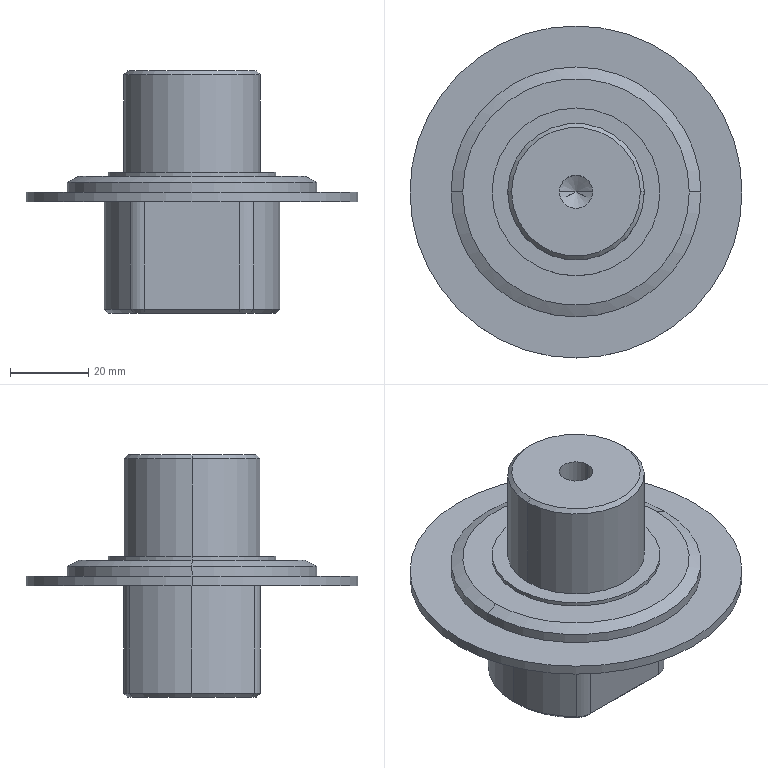Component | SolidWorks | 12AFixedFlatGrooveLargeWheel-EngravingAndMillingAxis-2_12ALargeStraighteningWheelAxis-1 | 1 solid | 52 faces | volume 86723 mm3 | cylinder 23 | cone 19 | plane 10 | commonest cylinder face diameters 8.5 x8 10 x4 45 x3 85 x2 64 x2 43 x2 35 x2 | material Q235